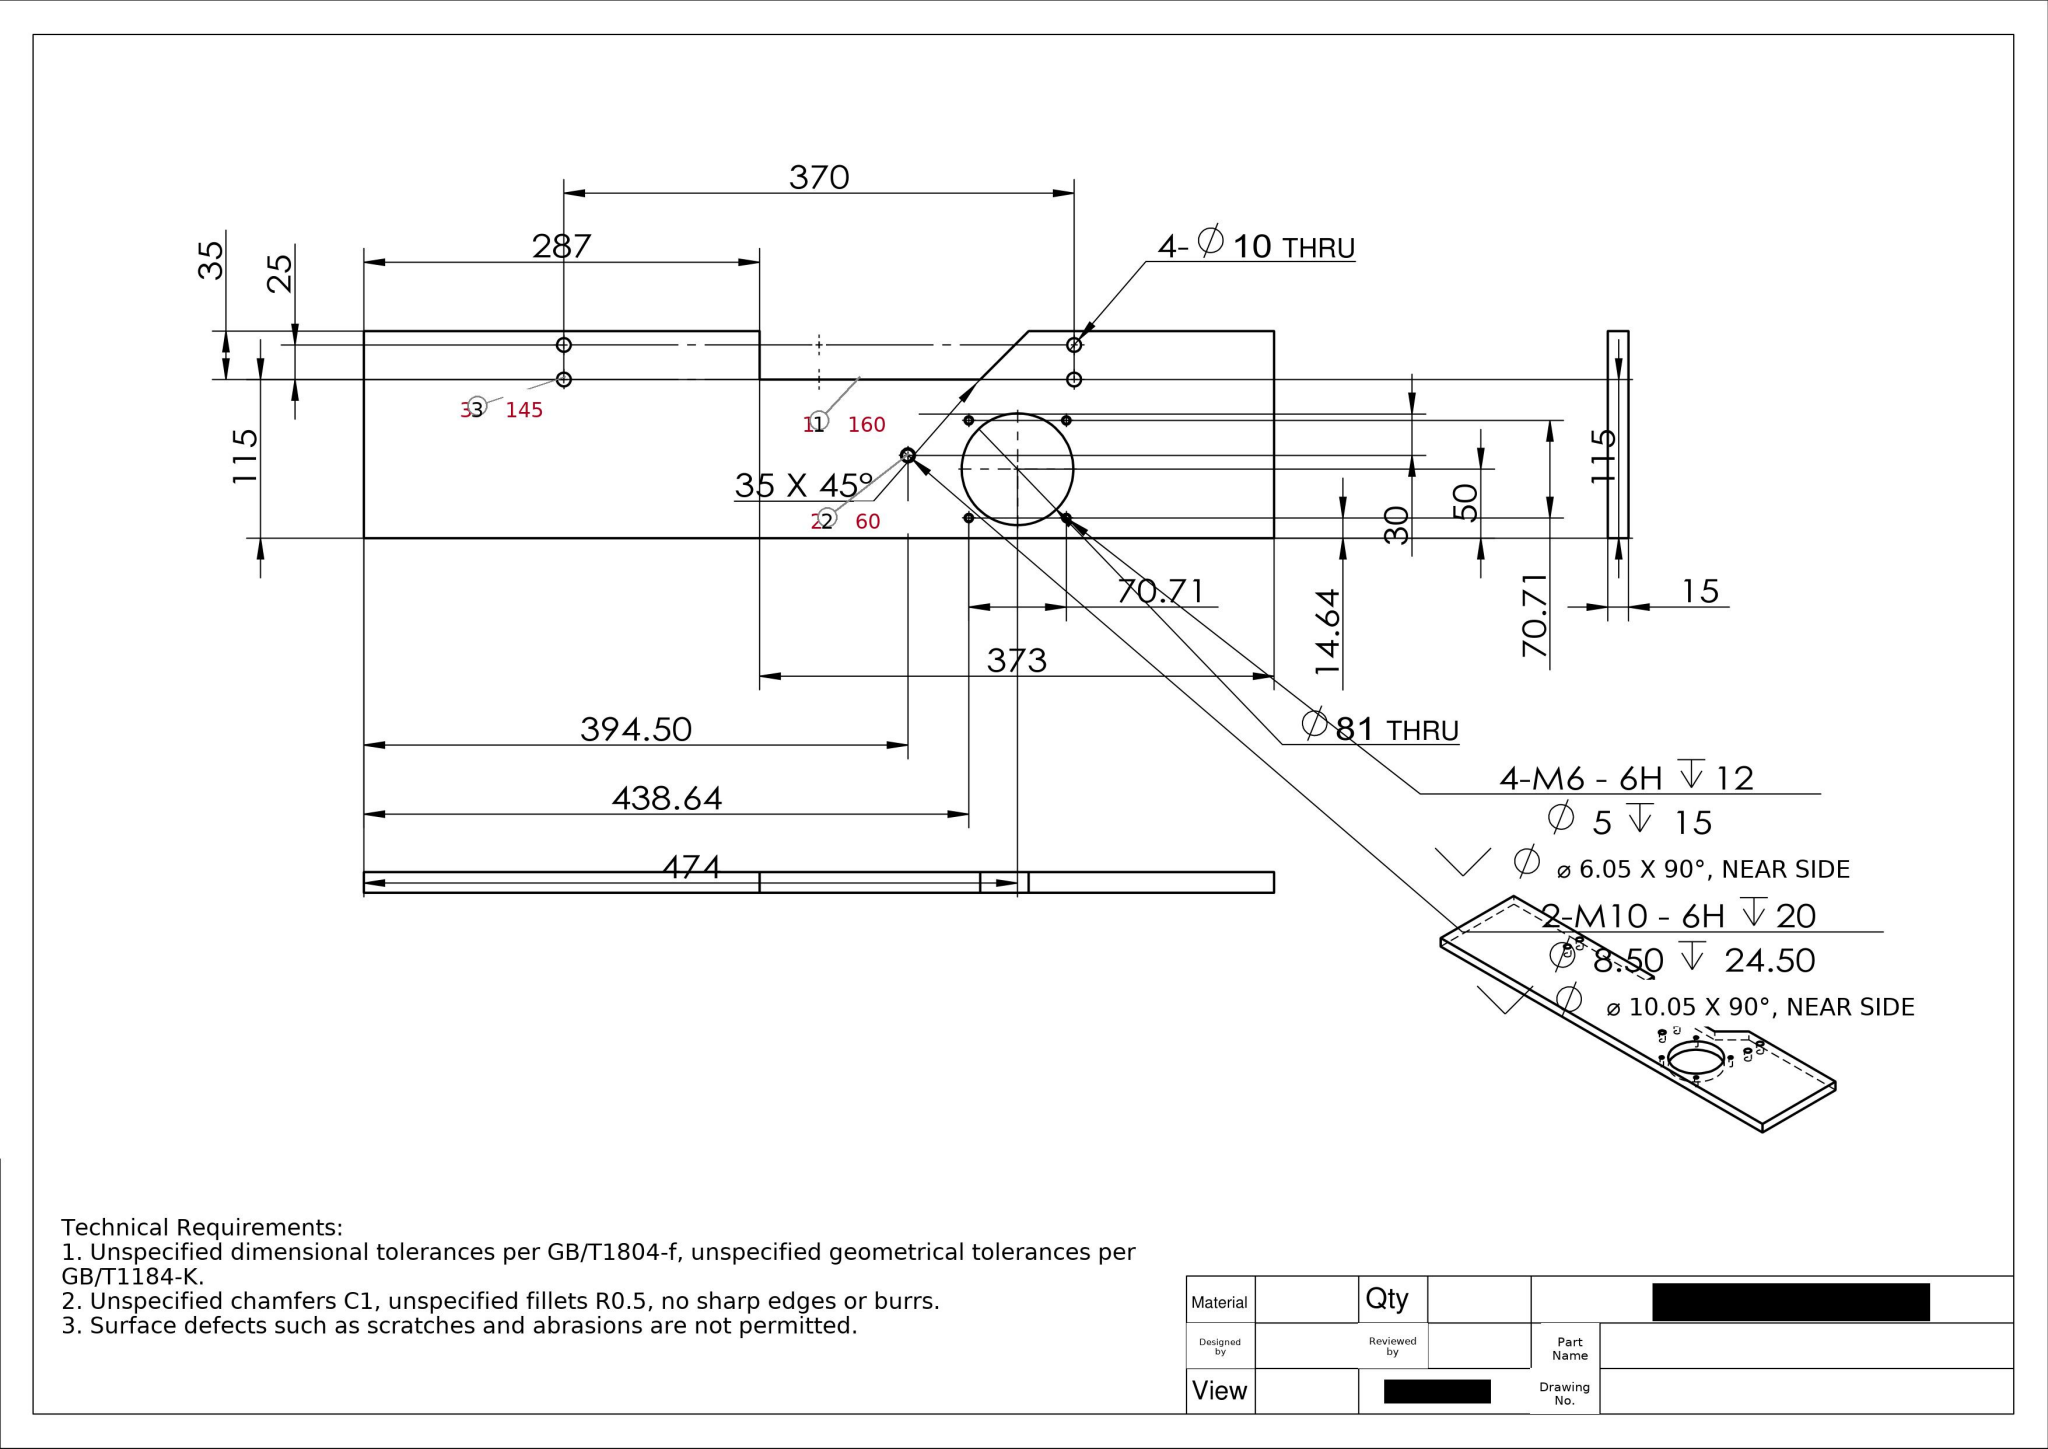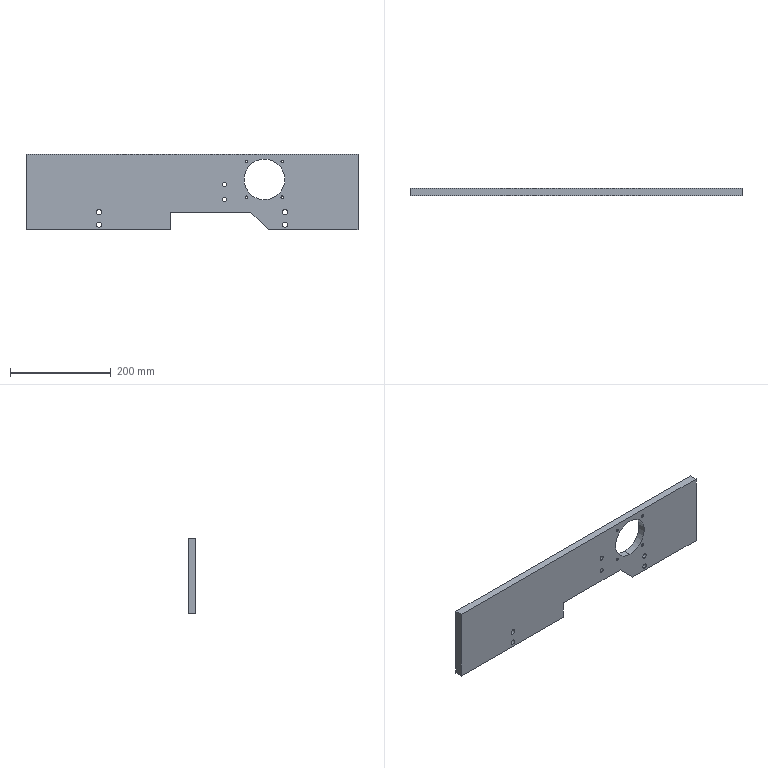Part | SolidWorks | mm | 1 solid | 44 faces | box 660 x 15 x 150 mm | volume 1306898 mm3 | cylinder 22 | cone 12 | plane 10 | commonest cylinder face diameters 5 x8 10 x8 8.5 x4 81 x2